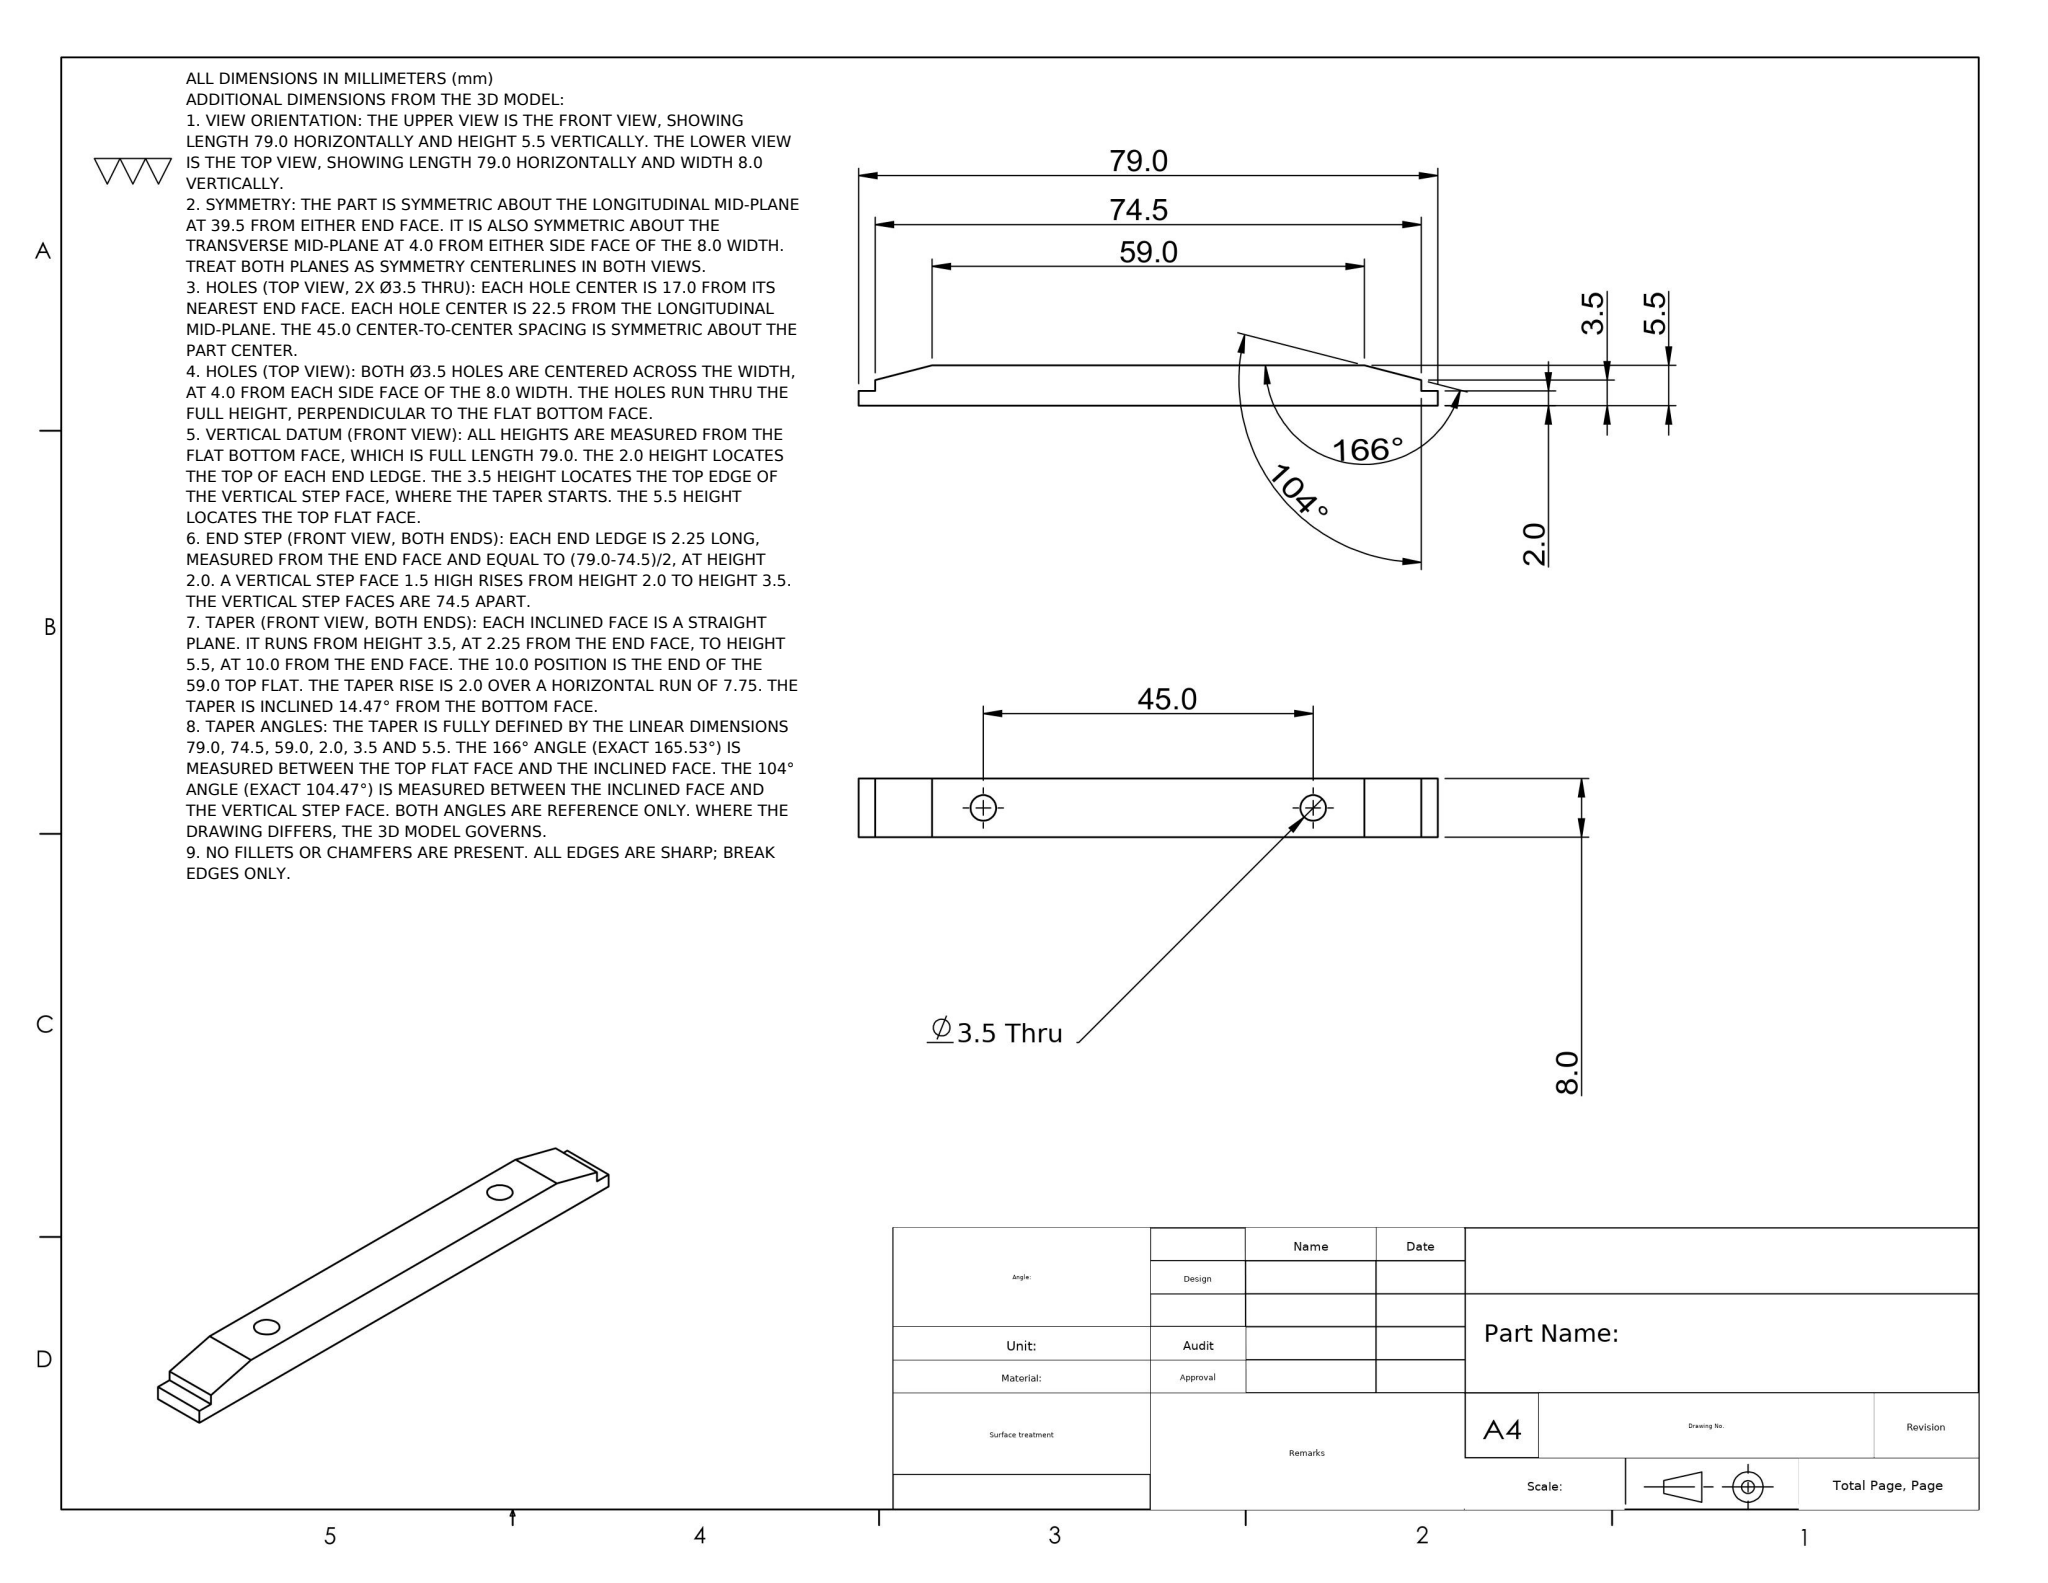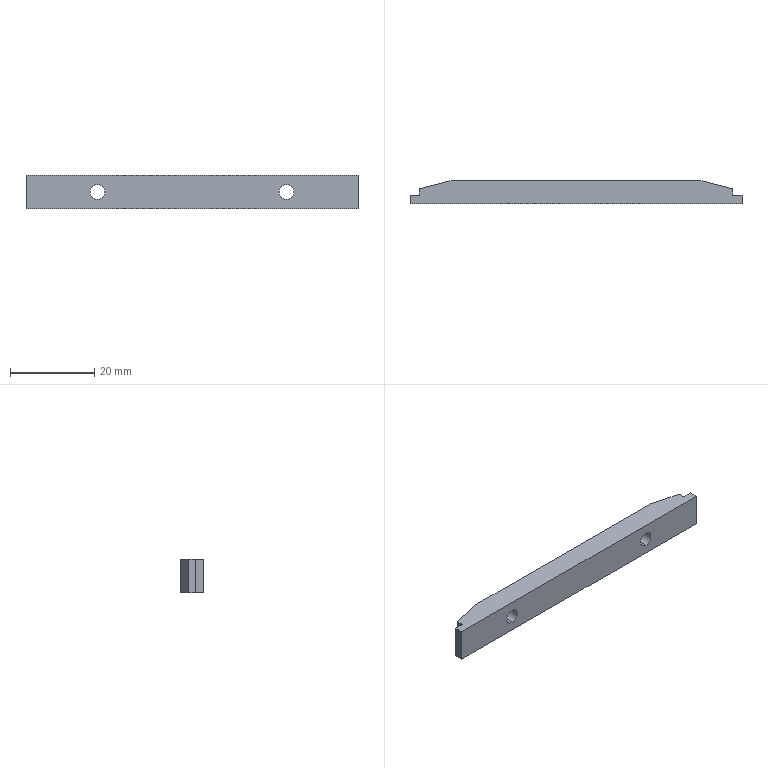Part | NX | mm | Tapered End Dual-Bore Mounting Bar | 1 solid | 16 faces | box 79 x 5.5 x 8 mm | volume 3120 mm3 | plane 12 | cylinder 4 | commonest cylinder face diameters 3.5 x4
STEP:
#1=COLOUR_RGB('',0.3961,0.8431,0.);
#2=FILL_AREA_STYLE_COLOUR('',#1);
#3=FILL_AREA_STYLE('',(#2));
#4=SURFACE_STYLE_FILL_AREA(#3);
#5=SURFACE_SIDE_STYLE('',(#4));
#6=SURFACE_STYLE_USAGE(.BOTH.,#5);
#7=PRESENTATION_STYLE_ASSIGNMENT((#6));
#8=CARTESIAN_POINT('',(22.5,-0.,2.25));
#9=VERTEX_POINT('',#8);
#10=CARTESIAN_POINT('',(22.5,-0.,5.75));
#11=VERTEX_POINT('',#10);
#12=CARTESIAN_POINT('',(22.5,-0.,4.));
#13=DIRECTION('',(0.,1.,0.));
#14=DIRECTION('',(0.,0.,1.));
#15=AXIS2_PLACEMENT_3D('',#12,#13,#14);
#16=CIRCLE('',#15,1.75);
#17=EDGE_CURVE('',#9,#11,#16,.T.);
#18=ORIENTED_EDGE('',*,*,#17,.F.);
#19=CARTESIAN_POINT('',(22.5,5.5,2.25));
#20=VERTEX_POINT('',#19);
#21=CARTESIAN_POINT('',(22.5,-0.,2.25));
#22=DIRECTION('',(0.,1.,0.));
#23=VECTOR('',#22,1000.);
#24=LINE('',#21,#23);
#25=EDGE_CURVE('',#9,#20,#24,.T.);
#26=ORIENTED_EDGE('',*,*,#25,.T.);
#27=CARTESIAN_POINT('',(22.5,5.5,5.75));
#28=VERTEX_POINT('',#27);
#29=CARTESIAN_POINT('',(22.5,5.5,4.));
#30=DIRECTION('',(0.,1.,0.));
#31=DIRECTION('',(0.,0.,1.));
#32=AXIS2_PLACEMENT_3D('',#29,#30,#31);
#33=CIRCLE('',#32,1.75);
#34=EDGE_CURVE('',#20,#28,#33,.T.);
#35=ORIENTED_EDGE('',*,*,#34,.T.);
#36=CARTESIAN_POINT('',(22.5,-0.,5.75));
#37=DIRECTION('',(0.,1.,0.));
#38=VECTOR('',#37,1000.);
#39=LINE('',#36,#38);
#40=EDGE_CURVE('',#11,#28,#39,.T.);
#41=ORIENTED_EDGE('',*,*,#40,.F.);
#42=EDGE_LOOP('',(#18,#26,#35,#41));
#43=FACE_OUTER_BOUND('',#42,.T.);
#44=CARTESIAN_POINT('',(22.5,-0.,4.));
#45=DIRECTION('',(0.,1.,0.));
#46=DIRECTION('',(0.,0.,1.));
#47=AXIS2_PLACEMENT_3D('',#44,#45,#46);
#48=CYLINDRICAL_SURFACE('',#47,1.75);
#49=ADVANCED_FACE('',(#43),#48,.F.);
#50=CARTESIAN_POINT('',(-22.5,-0.,2.25));
#51=VERTEX_POINT('',#50);
#52=CARTESIAN_POINT('',(-22.5,-0.,5.75));
#53=VERTEX_POINT('',#52);
#54=CARTESIAN_POINT('',(-22.5,-0.,4.));
#55=DIRECTION('',(0.,1.,0.));
#56=DIRECTION('',(0.,0.,1.));
#57=AXIS2_PLACEMENT_3D('',#54,#55,#56);
#58=CIRCLE('',#57,1.75);
#59=EDGE_CURVE('',#51,#53,#58,.T.);
#60=ORIENTED_EDGE('',*,*,#59,.F.);
#61=CARTESIAN_POINT('',(-22.5,5.5,2.25));
#62=VERTEX_POINT('',#61);
#63=CARTESIAN_POINT('',(-22.5,-0.,2.25));
#64=DIRECTION('',(0.,1.,0.));
#65=VECTOR('',#64,1000.);
#66=LINE('',#63,#65);
#67=EDGE_CURVE('',#51,#62,#66,.T.);
#68=ORIENTED_EDGE('',*,*,#67,.T.);
#69=CARTESIAN_POINT('',(-22.5,5.5,5.75));
#70=VERTEX_POINT('',#69);
#71=CARTESIAN_POINT('',(-22.5,5.5,4.));
#72=DIRECTION('',(0.,1.,0.));
#73=DIRECTION('',(0.,0.,1.));
#74=AXIS2_PLACEMENT_3D('',#71,#72,#73);
#75=CIRCLE('',#74,1.75);
#76=EDGE_CURVE('',#62,#70,#75,.T.);
#77=ORIENTED_EDGE('',*,*,#76,.T.);
#78=CARTESIAN_POINT('',(-22.5,-0.,5.75));
#79=DIRECTION('',(0.,1.,0.));
#80=VECTOR('',#79,1000.);
#81=LINE('',#78,#80);
#82=EDGE_CURVE('',#53,#70,#81,.T.);
#83=ORIENTED_EDGE('',*,*,#82,.F.);
#84=EDGE_LOOP('',(#60,#68,#77,#83));
#85=FACE_OUTER_BOUND('',#84,.T.);
#86=CARTESIAN_POINT('',(-22.5,-0.,4.));
#87=DIRECTION('',(0.,1.,0.));
#88=DIRECTION('',(0.,0.,1.));
#89=AXIS2_PLACEMENT_3D('',#86,#87,#88);
#90=CYLINDRICAL_SURFACE('',#89,1.75);
#91=ADVANCED_FACE('',(#85),#90,.F.);
#92=CARTESIAN_POINT('',(-39.5,2.,0.));
#93=VERTEX_POINT('',#92);
#94=CARTESIAN_POINT('',(-39.5,-0.,0.));
#95=VERTEX_POINT('',#94);
#96=CARTESIAN_POINT('',(-39.5,-0.,0.));
#97=DIRECTION('',(0.,-1.,0.));
#98=VECTOR('',#97,1000.);
#99=LINE('',#96,#98);
#100=EDGE_CURVE('',#93,#95,#99,.T.);
#101=ORIENTED_EDGE('',*,*,#100,.T.);
#102=CARTESIAN_POINT('',(-39.5,-0.,8.));
#103=VERTEX_POINT('',#102);
#104=CARTESIAN_POINT('',(-39.5,-0.,8.));
#105=DIRECTION('',(0.,0.,-1.));
#106=VECTOR('',#105,1000.);
#107=LINE('',#104,#106);
#108=EDGE_CURVE('',#103,#95,#107,.T.);
#109=ORIENTED_EDGE('',*,*,#108,.F.);
#110=CARTESIAN_POINT('',(-39.5,2.,8.));
#111=VERTEX_POINT('',#110);
#112=CARTESIAN_POINT('',(-39.5,-0.,8.));
#113=DIRECTION('',(0.,-1.,0.));
#114=VECTOR('',#113,1000.);
#115=LINE('',#112,#114);
#116=EDGE_CURVE('',#111,#103,#115,.T.);
#117=ORIENTED_EDGE('',*,*,#116,.F.);
#118=CARTESIAN_POINT('',(-39.5,2.,8.));
#119=DIRECTION('',(0.,0.,-1.));
#120=VECTOR('',#119,1000.);
#121=LINE('',#118,#120);
#122=EDGE_CURVE('',#111,#93,#121,.T.);
#123=ORIENTED_EDGE('',*,*,#122,.T.);
#124=EDGE_LOOP('',(#101,#109,#117,#123));
#125=FACE_OUTER_BOUND('',#124,.T.);
#126=CARTESIAN_POINT('',(-39.5,-0.,8.));
#127=DIRECTION('',(1.,0.,0.));
#128=DIRECTION('',(0.,0.,-1.));
#129=AXIS2_PLACEMENT_3D('',#126,#127,#128);
#130=PLANE('',#129);
#131=ADVANCED_FACE('',(#125),#130,.F.);
#132=CARTESIAN_POINT('',(22.5,-0.,4.));
#133=DIRECTION('',(0.,1.,0.));
#134=DIRECTION('',(0.,0.,1.));
#135=AXIS2_PLACEMENT_3D('',#132,#133,#134);
#136=CIRCLE('',#135,1.75);
#137=EDGE_CURVE('',#11,#9,#136,.T.);
#138=ORIENTED_EDGE('',*,*,#137,.T.);
#139=ORIENTED_EDGE('',*,*,#17,.T.);
#140=EDGE_LOOP('',(#138,#139));
#141=FACE_BOUND('',#140,.T.);
#142=CARTESIAN_POINT('',(-22.5,-0.,4.));
#143=DIRECTION('',(0.,1.,0.));
#144=DIRECTION('',(0.,0.,1.));
#145=AXIS2_PLACEMENT_3D('',#142,#143,#144);
#146=CIRCLE('',#145,1.75);
#147=EDGE_CURVE('',#53,#51,#146,.T.);
#148=ORIENTED_EDGE('',*,*,#147,.T.);
#149=ORIENTED_EDGE('',*,*,#59,.T.);
#150=EDGE_LOOP('',(#148,#149));
#151=FACE_BOUND('',#150,.T.);
#152=CARTESIAN_POINT('',(39.5,-0.,0.));
#153=VERTEX_POINT('',#152);
#154=CARTESIAN_POINT('',(39.5,-0.,0.));
#155=DIRECTION('',(1.,0.,0.));
#156=VECTOR('',#155,1000.);
#157=LINE('',#154,#156);
#158=EDGE_CURVE('',#95,#153,#157,.T.);
#159=ORIENTED_EDGE('',*,*,#158,.T.);
#160=CARTESIAN_POINT('',(39.5,-0.,8.));
#161=VERTEX_POINT('',#160);
#162=CARTESIAN_POINT('',(39.5,-0.,8.));
#163=DIRECTION('',(0.,0.,-1.));
#164=VECTOR('',#163,1000.);
#165=LINE('',#162,#164);
#166=EDGE_CURVE('',#161,#153,#165,.T.);
#167=ORIENTED_EDGE('',*,*,#166,.F.);
#168=CARTESIAN_POINT('',(39.5,-0.,8.));
#169=DIRECTION('',(1.,0.,0.));
#170=VECTOR('',#169,1000.);
#171=LINE('',#168,#170);
#172=EDGE_CURVE('',#103,#161,#171,.T.);
#173=ORIENTED_EDGE('',*,*,#172,.F.);
#174=ORIENTED_EDGE('',*,*,#108,.T.);
#175=EDGE_LOOP('',(#159,#167,#173,#174));
#176=FACE_OUTER_BOUND('',#175,.T.);
#177=CARTESIAN_POINT('',(39.5,-0.,8.));
#178=DIRECTION('',(0.,1.,0.));
#179=DIRECTION('',(0.,0.,1.));
#180=AXIS2_PLACEMENT_3D('',#177,#178,#179);
#181=PLANE('',#180);
#182=ADVANCED_FACE('',(#141,#151,#176),#181,.F.);
#183=CARTESIAN_POINT('',(39.5,2.,0.));
#184=VERTEX_POINT('',#183);
#185=CARTESIAN_POINT('',(39.5,-0.,0.));
#186=DIRECTION('',(0.,1.,0.));
#187=VECTOR('',#186,1000.);
#188=LINE('',#185,#187);
#189=EDGE_CURVE('',#153,#184,#188,.T.);
#190=ORIENTED_EDGE('',*,*,#189,.T.);
#191=CARTESIAN_POINT('',(39.5,2.,8.));
#192=VERTEX_POINT('',#191);
#193=CARTESIAN_POINT('',(39.5,2.,8.));
#194=DIRECTION('',(0.,0.,-1.));
#195=VECTOR('',#194,1000.);
#196=LINE('',#193,#195);
#197=EDGE_CURVE('',#192,#184,#196,.T.);
#198=ORIENTED_EDGE('',*,*,#197,.F.);
#199=CARTESIAN_POINT('',(39.5,-0.,8.));
#200=DIRECTION('',(0.,1.,0.));
#201=VECTOR('',#200,1000.);
#202=LINE('',#199,#201);
#203=EDGE_CURVE('',#161,#192,#202,.T.);
#204=ORIENTED_EDGE('',*,*,#203,.F.);
#205=ORIENTED_EDGE('',*,*,#166,.T.);
#206=EDGE_LOOP('',(#190,#198,#204,#205));
#207=FACE_OUTER_BOUND('',#206,.T.);
#208=CARTESIAN_POINT('',(39.5,-0.,8.));
#209=DIRECTION('',(-1.,0.,0.));
#210=DIRECTION('',(0.,0.,1.));
#211=AXIS2_PLACEMENT_3D('',#208,#209,#210);
#212=PLANE('',#211);
#213=ADVANCED_FACE('',(#207),#212,.F.);
#214=CARTESIAN_POINT('',(37.25,2.,0.));
#215=VERTEX_POINT('',#214);
#216=CARTESIAN_POINT('',(39.5,2.,0.));
#217=DIRECTION('',(-1.,0.,0.));
#218=VECTOR('',#217,1000.);
#219=LINE('',#216,#218);
#220=EDGE_CURVE('',#184,#215,#219,.T.);
#221=ORIENTED_EDGE('',*,*,#220,.T.);
#222=CARTESIAN_POINT('',(37.25,2.,8.));
#223=VERTEX_POINT('',#222);
#224=CARTESIAN_POINT('',(37.25,2.,8.));
#225=DIRECTION('',(0.,0.,-1.));
#226=VECTOR('',#225,1000.);
#227=LINE('',#224,#226);
#228=EDGE_CURVE('',#223,#215,#227,.T.);
#229=ORIENTED_EDGE('',*,*,#228,.F.);
#230=CARTESIAN_POINT('',(39.5,2.,8.));
#231=DIRECTION('',(-1.,0.,0.));
#232=VECTOR('',#231,1000.);
#233=LINE('',#230,#232);
#234=EDGE_CURVE('',#192,#223,#233,.T.);
#235=ORIENTED_EDGE('',*,*,#234,.F.);
#236=ORIENTED_EDGE('',*,*,#197,.T.);
#237=EDGE_LOOP('',(#221,#229,#235,#236));
#238=FACE_OUTER_BOUND('',#237,.T.);
#239=CARTESIAN_POINT('',(39.5,2.,8.));
#240=DIRECTION('',(0.,-1.,0.));
#241=DIRECTION('',(0.,0.,-1.));
#242=AXIS2_PLACEMENT_3D('',#239,#240,#241);
#243=PLANE('',#242);
#244=ADVANCED_FACE('',(#238),#243,.F.);
#245=CARTESIAN_POINT('',(37.25,3.5,0.));
#246=VERTEX_POINT('',#245);
#247=CARTESIAN_POINT('',(37.25,2.,0.));
#248=DIRECTION('',(0.,1.,0.));
#249=VECTOR('',#248,1000.);
#250=LINE('',#247,#249);
#251=EDGE_CURVE('',#215,#246,#250,.T.);
#252=ORIENTED_EDGE('',*,*,#251,.T.);
#253=CARTESIAN_POINT('',(37.25,3.5,8.));
#254=VERTEX_POINT('',#253);
#255=CARTESIAN_POINT('',(37.25,3.5,8.));
#256=DIRECTION('',(0.,0.,-1.));
#257=VECTOR('',#256,1000.);
#258=LINE('',#255,#257);
#259=EDGE_CURVE('',#254,#246,#258,.T.);
#260=ORIENTED_EDGE('',*,*,#259,.F.);
#261=CARTESIAN_POINT('',(37.25,2.,8.));
#262=DIRECTION('',(0.,1.,0.));
#263=VECTOR('',#262,1000.);
#264=LINE('',#261,#263);
#265=EDGE_CURVE('',#223,#254,#264,.T.);
#266=ORIENTED_EDGE('',*,*,#265,.F.);
#267=ORIENTED_EDGE('',*,*,#228,.T.);
#268=EDGE_LOOP('',(#252,#260,#266,#267));
#269=FACE_OUTER_BOUND('',#268,.T.);
#270=CARTESIAN_POINT('',(37.25,2.,8.));
#271=DIRECTION('',(-1.,0.,0.));
#272=DIRECTION('',(0.,0.,1.));
#273=AXIS2_PLACEMENT_3D('',#270,#271,#272);
#274=PLANE('',#273);
#275=ADVANCED_FACE('',(#269),#274,.F.);
#276=CARTESIAN_POINT('',(29.5,5.5,0.));
#277=VERTEX_POINT('',#276);
#278=CARTESIAN_POINT('',(37.25,3.5,0.));
#279=DIRECTION('',(-0.9683,0.2499,0.));
#280=VECTOR('',#279,1000.);
#281=LINE('',#278,#280);
#282=EDGE_CURVE('',#246,#277,#281,.T.);
#283=ORIENTED_EDGE('',*,*,#282,.T.);
#284=CARTESIAN_POINT('',(29.5,5.5,8.));
#285=VERTEX_POINT('',#284);
#286=CARTESIAN_POINT('',(29.5,5.5,8.));
#287=DIRECTION('',(0.,0.,-1.));
#288=VECTOR('',#287,1000.);
#289=LINE('',#286,#288);
#290=EDGE_CURVE('',#285,#277,#289,.T.);
#291=ORIENTED_EDGE('',*,*,#290,.F.);
#292=CARTESIAN_POINT('',(37.25,3.5,8.));
#293=DIRECTION('',(-0.9683,0.2499,0.));
#294=VECTOR('',#293,1000.);
#295=LINE('',#292,#294);
#296=EDGE_CURVE('',#254,#285,#295,.T.);
#297=ORIENTED_EDGE('',*,*,#296,.F.);
#298=ORIENTED_EDGE('',*,*,#259,.T.);
#299=EDGE_LOOP('',(#283,#291,#297,#298));
#300=FACE_OUTER_BOUND('',#299,.T.);
#301=CARTESIAN_POINT('',(37.25,3.5,8.));
#302=DIRECTION('',(-0.2499,-0.9683,0.));
#303=DIRECTION('',(0.9683,-0.2499,0.));
#304=AXIS2_PLACEMENT_3D('',#301,#302,#303);
#305=PLANE('',#304);
#306=ADVANCED_FACE('',(#300),#305,.F.);
#307=CARTESIAN_POINT('',(22.5,5.5,4.));
#308=DIRECTION('',(0.,1.,0.));
#309=DIRECTION('',(0.,0.,1.));
#310=AXIS2_PLACEMENT_3D('',#307,#308,#309);
#311=CIRCLE('',#310,1.75);
#312=EDGE_CURVE('',#28,#20,#311,.T.);
#313=ORIENTED_EDGE('',*,*,#312,.F.);
#314=ORIENTED_EDGE('',*,*,#34,.F.);
#315=EDGE_LOOP('',(#313,#314));
#316=FACE_BOUND('',#315,.T.);
#317=CARTESIAN_POINT('',(-22.5,5.5,4.));
#318=DIRECTION('',(0.,1.,0.));
#319=DIRECTION('',(0.,0.,1.));
#320=AXIS2_PLACEMENT_3D('',#317,#318,#319);
#321=CIRCLE('',#320,1.75);
#322=EDGE_CURVE('',#70,#62,#321,.T.);
#323=ORIENTED_EDGE('',*,*,#322,.F.);
#324=ORIENTED_EDGE('',*,*,#76,.F.);
#325=EDGE_LOOP('',(#323,#324));
#326=FACE_BOUND('',#325,.T.);
#327=CARTESIAN_POINT('',(-29.5,5.5,0.));
#328=VERTEX_POINT('',#327);
#329=CARTESIAN_POINT('',(-29.5,5.5,0.));
#330=DIRECTION('',(-1.,0.,0.));
#331=VECTOR('',#330,1000.);
#332=LINE('',#329,#331);
#333=EDGE_CURVE('',#277,#328,#332,.T.);
#334=ORIENTED_EDGE('',*,*,#333,.T.);
#335=CARTESIAN_POINT('',(-29.5,5.5,8.));
#336=VERTEX_POINT('',#335);
#337=CARTESIAN_POINT('',(-29.5,5.5,8.));
#338=DIRECTION('',(0.,0.,-1.));
#339=VECTOR('',#338,1000.);
#340=LINE('',#337,#339);
#341=EDGE_CURVE('',#336,#328,#340,.T.);
#342=ORIENTED_EDGE('',*,*,#341,.F.);
#343=CARTESIAN_POINT('',(-29.5,5.5,8.));
#344=DIRECTION('',(-1.,0.,0.));
#345=VECTOR('',#344,1000.);
#346=LINE('',#343,#345);
#347=EDGE_CURVE('',#285,#336,#346,.T.);
#348=ORIENTED_EDGE('',*,*,#347,.F.);
#349=ORIENTED_EDGE('',*,*,#290,.T.);
#350=EDGE_LOOP('',(#334,#342,#348,#349));
#351=FACE_OUTER_BOUND('',#350,.T.);
#352=CARTESIAN_POINT('',(-29.5,5.5,8.));
#353=DIRECTION('',(0.,-1.,0.));
#354=DIRECTION('',(0.,0.,-1.));
#355=AXIS2_PLACEMENT_3D('',#352,#353,#354);
#356=PLANE('',#355);
#357=ADVANCED_FACE('',(#316,#326,#351),#356,.F.);
#358=CARTESIAN_POINT('',(-37.25,3.5,0.));
#359=VERTEX_POINT('',#358);
#360=CARTESIAN_POINT('',(-37.25,3.5,0.));
#361=DIRECTION('',(-0.9683,-0.2499,0.));
#362=VECTOR('',#361,1000.);
#363=LINE('',#360,#362);
#364=EDGE_CURVE('',#328,#359,#363,.T.);
#365=ORIENTED_EDGE('',*,*,#364,.T.);
#366=CARTESIAN_POINT('',(-37.25,3.5,8.));
#367=VERTEX_POINT('',#366);
#368=CARTESIAN_POINT('',(-37.25,3.5,8.));
#369=DIRECTION('',(0.,0.,-1.));
#370=VECTOR('',#369,1000.);
#371=LINE('',#368,#370);
#372=EDGE_CURVE('',#367,#359,#371,.T.);
#373=ORIENTED_EDGE('',*,*,#372,.F.);
#374=CARTESIAN_POINT('',(-37.25,3.5,8.));
#375=DIRECTION('',(-0.9683,-0.2499,0.));
#376=VECTOR('',#375,1000.);
#377=LINE('',#374,#376);
#378=EDGE_CURVE('',#336,#367,#377,.T.);
#379=ORIENTED_EDGE('',*,*,#378,.F.);
#380=ORIENTED_EDGE('',*,*,#341,.T.);
#381=EDGE_LOOP('',(#365,#373,#379,#380));
#382=FACE_OUTER_BOUND('',#381,.T.);
#383=CARTESIAN_POINT('',(-37.25,3.5,8.));
#384=DIRECTION('',(0.2499,-0.9683,0.));
#385=DIRECTION('',(0.9683,0.2499,0.));
#386=AXIS2_PLACEMENT_3D('',#383,#384,#385);
#387=PLANE('',#386);
#388=ADVANCED_FACE('',(#382),#387,.F.);
#389=CARTESIAN_POINT('',(-37.25,2.,0.));
#390=VERTEX_POINT('',#389);
#391=CARTESIAN_POINT('',(-37.25,2.,0.));
#392=DIRECTION('',(0.,-1.,0.));
#393=VECTOR('',#392,1000.);
#394=LINE('',#391,#393);
#395=EDGE_CURVE('',#359,#390,#394,.T.);
#396=ORIENTED_EDGE('',*,*,#395,.T.);
#397=CARTESIAN_POINT('',(-37.25,2.,8.));
#398=VERTEX_POINT('',#397);
#399=CARTESIAN_POINT('',(-37.25,2.,8.));
#400=DIRECTION('',(0.,0.,-1.));
#401=VECTOR('',#400,1000.);
#402=LINE('',#399,#401);
#403=EDGE_CURVE('',#398,#390,#402,.T.);
#404=ORIENTED_EDGE('',*,*,#403,.F.);
#405=CARTESIAN_POINT('',(-37.25,2.,8.));
#406=DIRECTION('',(0.,-1.,0.));
#407=VECTOR('',#406,1000.);
#408=LINE('',#405,#407);
#409=EDGE_CURVE('',#367,#398,#408,.T.);
#410=ORIENTED_EDGE('',*,*,#409,.F.);
#411=ORIENTED_EDGE('',*,*,#372,.T.);
#412=EDGE_LOOP('',(#396,#404,#410,#411));
#413=FACE_OUTER_BOUND('',#412,.T.);
#414=CARTESIAN_POINT('',(-37.25,2.,8.));
#415=DIRECTION('',(1.,0.,0.));
#416=DIRECTION('',(0.,0.,-1.));
#417=AXIS2_PLACEMENT_3D('',#414,#415,#416);
#418=PLANE('',#417);
#419=ADVANCED_FACE('',(#413),#418,.F.);
#420=CARTESIAN_POINT('',(-39.5,2.,0.));
#421=DIRECTION('',(-1.,0.,0.));
#422=VECTOR('',#421,1000.);
#423=LINE('',#420,#422);
#424=EDGE_CURVE('',#390,#93,#423,.T.);
#425=ORIENTED_EDGE('',*,*,#424,.T.);
#426=ORIENTED_EDGE('',*,*,#122,.F.);
#427=CARTESIAN_POINT('',(-39.5,2.,8.));
#428=DIRECTION('',(-1.,0.,0.));
#429=VECTOR('',#428,1000.);
#430=LINE('',#427,#429);
#431=EDGE_CURVE('',#398,#111,#430,.T.);
#432=ORIENTED_EDGE('',*,*,#431,.F.);
#433=ORIENTED_EDGE('',*,*,#403,.T.);
#434=EDGE_LOOP('',(#425,#426,#432,#433));
#435=FACE_OUTER_BOUND('',#434,.T.);
#436=CARTESIAN_POINT('',(-39.5,2.,8.));
#437=DIRECTION('',(0.,-1.,0.));
#438=DIRECTION('',(0.,0.,-1.));
#439=AXIS2_PLACEMENT_3D('',#436,#437,#438);
#440=PLANE('',#439);
#441=ADVANCED_FACE('',(#435),#440,.F.);
#442=ORIENTED_EDGE('',*,*,#116,.T.);
#443=ORIENTED_EDGE('',*,*,#172,.T.);
#444=ORIENTED_EDGE('',*,*,#203,.T.);
#445=ORIENTED_EDGE('',*,*,#234,.T.);
#446=ORIENTED_EDGE('',*,*,#265,.T.);
#447=ORIENTED_EDGE('',*,*,#296,.T.);
#448=ORIENTED_EDGE('',*,*,#347,.T.);
#449=ORIENTED_EDGE('',*,*,#378,.T.);
#450=ORIENTED_EDGE('',*,*,#409,.T.);
#451=ORIENTED_EDGE('',*,*,#431,.T.);
#452=EDGE_LOOP('',(#442,#443,#444,#445,#446,#447,#448,#449,#450,#451));
#453=FACE_OUTER_BOUND('',#452,.T.);
#454=CARTESIAN_POINT('',(-39.5,2.,8.));
#455=DIRECTION('',(0.,0.,-1.));
#456=DIRECTION('',(-1.,0.,0.));
#457=AXIS2_PLACEMENT_3D('',#454,#455,#456);
#458=PLANE('',#457);
#459=ADVANCED_FACE('',(#453),#458,.F.);
#460=ORIENTED_EDGE('',*,*,#100,.F.);
#461=ORIENTED_EDGE('',*,*,#424,.F.);
#462=ORIENTED_EDGE('',*,*,#395,.F.);
#463=ORIENTED_EDGE('',*,*,#364,.F.);
#464=ORIENTED_EDGE('',*,*,#333,.F.);
#465=ORIENTED_EDGE('',*,*,#282,.F.);
#466=ORIENTED_EDGE('',*,*,#251,.F.);
#467=ORIENTED_EDGE('',*,*,#220,.F.);
#468=ORIENTED_EDGE('',*,*,#189,.F.);
#469=ORIENTED_EDGE('',*,*,#158,.F.);
#470=EDGE_LOOP('',(#460,#461,#462,#463,#464,#465,#466,#467,#468,#469));
#471=FACE_OUTER_BOUND('',#470,.T.);
#472=CARTESIAN_POINT('',(-39.5,2.,0.));
#473=DIRECTION('',(0.,0.,-1.));
#474=DIRECTION('',(-1.,0.,0.));
#475=AXIS2_PLACEMENT_3D('',#472,#473,#474);
#476=PLANE('',#475);
#477=ADVANCED_FACE('',(#471),#476,.T.);
#478=ORIENTED_EDGE('',*,*,#67,.F.);
#479=ORIENTED_EDGE('',*,*,#147,.F.);
#480=ORIENTED_EDGE('',*,*,#82,.T.);
#481=ORIENTED_EDGE('',*,*,#322,.T.);
#482=EDGE_LOOP('',(#478,#479,#480,#481));
#483=FACE_OUTER_BOUND('',#482,.T.);
#484=CARTESIAN_POINT('',(-22.5,-0.,4.));
#485=DIRECTION('',(0.,1.,0.));
#486=DIRECTION('',(0.,0.,1.));
#487=AXIS2_PLACEMENT_3D('',#484,#485,#486);
#488=CYLINDRICAL_SURFACE('',#487,1.75);
#489=ADVANCED_FACE('',(#483),#488,.F.);
#490=ORIENTED_EDGE('',*,*,#25,.F.);
#491=ORIENTED_EDGE('',*,*,#137,.F.);
#492=ORIENTED_EDGE('',*,*,#40,.T.);
#493=ORIENTED_EDGE('',*,*,#312,.T.);
#494=EDGE_LOOP('',(#490,#491,#492,#493));
#495=FACE_OUTER_BOUND('',#494,.T.);
#496=CARTESIAN_POINT('',(22.5,-0.,4.));
#497=DIRECTION('',(0.,1.,0.));
#498=DIRECTION('',(0.,0.,1.));
#499=AXIS2_PLACEMENT_3D('',#496,#497,#498);
#500=CYLINDRICAL_SURFACE('',#499,1.75);
#501=ADVANCED_FACE('',(#495),#500,.F.);
#502=CLOSED_SHELL('',(#49,#91,#131,#182,#213,#244,#275,#306,#357,#388,#419,#441,#459,#477,#489,#501));
#503=MANIFOLD_SOLID_BREP('',#502);
#504=STYLED_ITEM('',(#7),#503);
#505=PRESENTATION_LAYER_ASSIGNMENT('','',(#504));
#506=(LENGTH_UNIT()NAMED_UNIT(*)SI_UNIT(.MILLI.,.METRE.));
#507=UNCERTAINTY_MEASURE_WITH_UNIT(LENGTH_MEASURE(0.00001),#506,'','');
#508=(NAMED_UNIT(*)PLANE_ANGLE_UNIT()SI_UNIT($,.RADIAN.));
#509=(NAMED_UNIT(*)SI_UNIT($,.STERADIAN.)SOLID_ANGLE_UNIT());
#510=(GEOMETRIC_REPRESENTATION_CONTEXT(3)GLOBAL_UNCERTAINTY_ASSIGNED_CONTEXT((#507))GLOBAL_UNIT_ASSIGNED_CONTEXT((#506,#508,#509))REPRESENTATION_CONTEXT('',''));
#511=MECHANICAL_DESIGN_GEOMETRIC_PRESENTATION_REPRESENTATION('',(#504),#510);
#512=COLOUR_RGB('',0.3961,0.8431,0.);
#513=FILL_AREA_STYLE_COLOUR('',#512);
#514=FILL_AREA_STYLE('',(#513));
#515=SURFACE_STYLE_FILL_AREA(#514);
#516=SURFACE_SIDE_STYLE('',(#515));
#517=SURFACE_STYLE_USAGE(.BOTH.,#516);
#518=PRESENTATION_STYLE_ASSIGNMENT((#517));
#519=CARTESIAN_POINT('',(0.,0.,0.));
#520=DIRECTION('',(0.,0.,1.));
#521=DIRECTION('',(1.,0.,0.));
#522=AXIS2_PLACEMENT_3D('',#519,#520,#521);
#523=(LENGTH_UNIT()NAMED_UNIT(*)SI_UNIT(.MILLI.,.METRE.));
#524=UNCERTAINTY_MEASURE_WITH_UNIT(LENGTH_MEASURE(0.00001),#523,'','');
#525=(NAMED_UNIT(*)PLANE_ANGLE_UNIT()SI_UNIT($,.RADIAN.));
#526=(NAMED_UNIT(*)SI_UNIT($,.STERADIAN.)SOLID_ANGLE_UNIT());
#527=(GEOMETRIC_REPRESENTATION_CONTEXT(3)GLOBAL_UNCERTAINTY_ASSIGNED_CONTEXT((#524))GLOBAL_UNIT_ASSIGNED_CONTEXT((#523,#525,#526))REPRESENTATION_CONTEXT('',''));
#528=ADVANCED_BREP_SHAPE_REPRESENTATION('',(#503,#522),#527);
#529=STYLED_ITEM('',(#518),#528);
#530=PRESENTATION_LAYER_ASSIGNMENT('','',(#529));
#531=(LENGTH_UNIT()NAMED_UNIT(*)SI_UNIT(.MILLI.,.METRE.));
#532=UNCERTAINTY_MEASURE_WITH_UNIT(LENGTH_MEASURE(0.00001),#531,'','');
#533=(NAMED_UNIT(*)PLANE_ANGLE_UNIT()SI_UNIT($,.RADIAN.));
#534=(NAMED_UNIT(*)SI_UNIT($,.STERADIAN.)SOLID_ANGLE_UNIT());
#535=(GEOMETRIC_REPRESENTATION_CONTEXT(3)GLOBAL_UNCERTAINTY_ASSIGNED_CONTEXT((#532))GLOBAL_UNIT_ASSIGNED_CONTEXT((#531,#533,#534))REPRESENTATION_CONTEXT('',''));
#536=MECHANICAL_DESIGN_GEOMETRIC_PRESENTATION_REPRESENTATION('',(#529),#535);